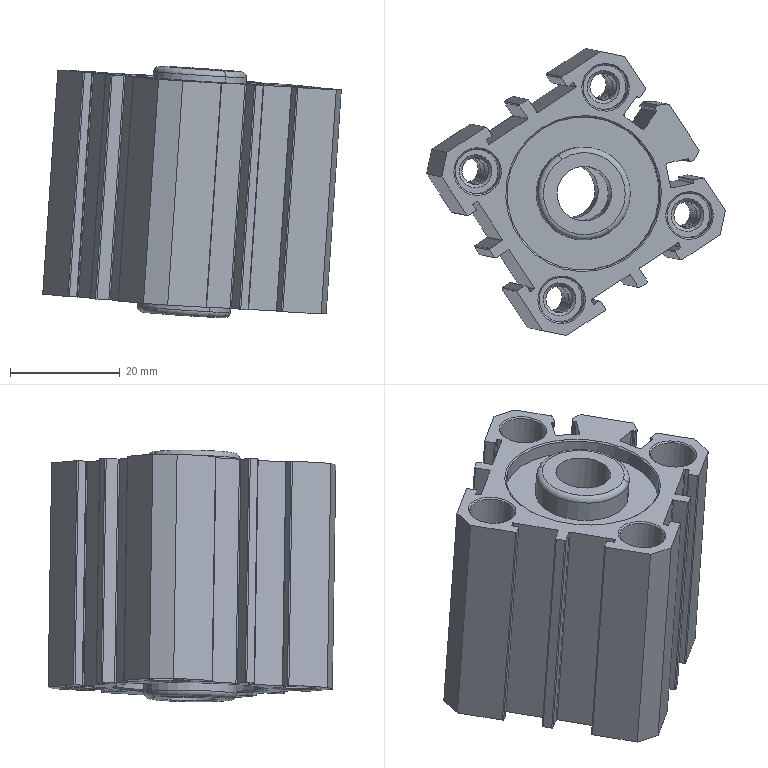Component | SolidWorks | SDAJ25x20-20B(00)+()-1_SDAJ-25x20_20b-1 | 1 solid | 245 faces | box 54.53 x 52.51 x 45.94 mm | volume 37343 mm3 | cylinder 111 | plane 86 | cone 44 | torus 4 | commonest cylinder face diameters 0.4 x46 8.2 x16 4.917 x16 4.6 x8 0.8 x7 17 x4 28 x4 4.134 x4
build123d program:
from build123d import *

# Parameters (mm, degrees)
BOSS_EXTRUDE1_DEPTH  = 41
LPATTERN1_COUNT      = 2
LPATTERN1_PITCH      = 28
LPATTERN1_COUNT_DIR2 = 2
LPATTERN1_PITCH_DIR2 = 28
LPATTERN2_COUNT      = 2
LPATTERN2_PITCH      = 28
LPATTERN2_COUNT_DIR2 = 2
LPATTERN2_PITCH_DIR2 = 28
HOLE1_D              = 4.134
HOLE1_DEPTH          = 6
HOLE1_CSINK_D        = 5
HOLE1_CSINK_ANGLE    = 90
HOLE1_TIP            = 1.193
HOLE2_D              = 4.134
HOLE2_DEPTH          = 6
HOLE2_CSINK_D        = 5
HOLE2_CSINK_ANGLE    = 90
HOLE2_TIP            = 1.193


with BuildPart() as part:
    # Sketch1 → Boss-Extrude1 (new body)
    with BuildSketch(Plane(origin=(0, 0, 0), x_dir=(0, 0, -1), z_dir=(1, 0, 0))):
        with BuildLine():
            Line((-20, 16.8), (-20, 8.4))
            ThreePointArc((-20, 8.4), (-19.941, 8.259), (-19.8, 8.2))
            Line((-19.8, 8.2), (-18.2, 8.2))
            ThreePointArc((-18.2, 8.2), (-18.059, 8.259), (-18, 8.4))
            Line((-18, 8.4), (-18, 9.4))
            ThreePointArc((-18, 9.4), (-17.941, 9.541), (-17.8, 9.6))
            Line((-17.8, 9.6), (-17.2, 9.6))
            ThreePointArc((-17.2, 9.6), (-17.059, 9.541), (-17, 9.4))
            Line((-17, 9.4), (-17, 1.2))
            ThreePointArc((-17, 1.2), (-17.059, 1.059), (-17.2, 1))
            Line((-17.2, 1), (-19.8, 1))
            ThreePointArc((-19.8, 1), (-19.941, 0.9414), (-20, 0.8))
            Line((-20, 0.8), (-20, -0.8))
            ThreePointArc((-20, -0.8), (-19.941, -0.9414), (-19.8, -1))
            Line((-19.8, -1), (-17.2, -1))
            ThreePointArc((-17.2, -1), (-17.059, -1.059), (-17, -1.2))
            Line((-17, -1.2), (-17, -9.4))
            ThreePointArc((-17, -9.4), (-17.059, -9.541), (-17.2, -9.6))
            Line((-17.2, -9.6), (-17.8, -9.6))
            ThreePointArc((-17.8, -9.6), (-17.941, -9.541), (-18, -9.4))
            Line((-18, -9.4), (-18, -8.4))
            ThreePointArc((-18, -8.4), (-18.059, -8.259), (-18.2, -8.2))
            Line((-18.2, -8.2), (-19.8, -8.2))
            ThreePointArc((-19.8, -8.2), (-19.941, -8.259), (-20, -8.4))
            Line((-20, -8.4), (-20, -16.8))
            Line((-20, -16.8), (-16.8, -20))
            Line((-16.8, -20), (-8.4, -20))
            ThreePointArc((-8.4, -20), (-8.259, -19.941), (-8.2, -19.8))
            Line((-8.2, -19.8), (-8.2, -18.2))
            ThreePointArc((-8.2, -18.2), (-8.259, -18.059), (-8.4, -18))
            Line((-8.4, -18), (-9.4, -18))
            ThreePointArc((-9.4, -18), (-9.541, -17.941), (-9.6, -17.8))
            Line((-9.6, -17.8), (-9.6, -17.2))
            ThreePointArc((-9.6, -17.2), (-9.541, -17.059), (-9.4, -17))
            Line((-9.4, -17), (-1.2, -17))
            ThreePointArc((-1.2, -17), (-1.059, -17.059), (-1, -17.2))
            Line((-1, -17.2), (-1, -19.8))
            ThreePointArc((-1, -19.8), (-0.9414, -19.941), (-0.8, -20))
            Line((-0.8, -20), (0.8, -20))
            ThreePointArc((0.8, -20), (0.9414, -19.941), (1, -19.8))
            Line((1, -19.8), (1, -17.2))
            ThreePointArc((1, -17.2), (1.059, -17.059), (1.2, -17))
            Line((1.2, -17), (9.4, -17))
            ThreePointArc((9.4, -17), (9.541, -17.059), (9.6, -17.2))
            Line((9.6, -17.2), (9.6, -17.8))
            ThreePointArc((9.6, -17.8), (9.541, -17.941), (9.4, -18))
            Line((9.4, -18), (8.4, -18))
            ThreePointArc((8.4, -18), (8.259, -18.059), (8.2, -18.2))
            Line((8.2, -18.2), (8.2, -19.8))
            ThreePointArc((8.2, -19.8), (8.259, -19.941), (8.4, -20))
            Line((8.4, -20), (16.8, -20))
            Line((16.8, -20), (20, -16.8))
            Line((20, -16.8), (20, -8.4))
            ThreePointArc((20, -8.4), (19.941, -8.259), (19.8, -8.2))
            Line((19.8, -8.2), (18.2, -8.2))
            ThreePointArc((18.2, -8.2), (18.059, -8.259), (18, -8.4))
            Line((18, -8.4), (18, -9.4))
            ThreePointArc((18, -9.4), (17.941, -9.541), (17.8, -9.6))
            Line((17.8, -9.6), (17.2, -9.6))
            ThreePointArc((17.2, -9.6), (17.059, -9.541), (17, -9.4))
            Line((17, -9.4), (17, -1.2))
            ThreePointArc((17, -1.2), (17.059, -1.059), (17.2, -1))
            Line((17.2, -1), (19.8, -1))
            ThreePointArc((19.8, -1), (19.941, -0.9414), (20, -0.8))
            Line((20, -0.8), (20, 0.8))
            ThreePointArc((20, 0.8), (19.941, 0.9414), (19.8, 1))
            Line((19.8, 1), (17.2, 1))
            ThreePointArc((17.2, 1), (17.059, 1.059), (17, 1.2))
            Line((17, 1.2), (17, 9.4))
            ThreePointArc((17, 9.4), (17.059, 9.541), (17.2, 9.6))
            Line((17.2, 9.6), (17.8, 9.6))
            ThreePointArc((17.8, 9.6), (17.941, 9.541), (18, 9.4))
            Line((18, 9.4), (18, 8.4))
            ThreePointArc((18, 8.4), (18.059, 8.259), (18.2, 8.2))
            Line((18.2, 8.2), (19.8, 8.2))
            ThreePointArc((19.8, 8.2), (19.941, 8.259), (20, 8.4))
            Line((20, 8.4), (20, 16.8))
            Line((20, 16.8), (16.8, 20))
            Line((16.8, 20), (9.978, 20))
            ThreePointArc((9.978, 20), (9.753, 19.931), (9.606, 19.747))
            Line((9.606, 19.747), (9.022, 18.264))
            ThreePointArc((9.022, 18.264), (9.024, 18.111), (9.134, 18.005))
            Line((9.134, 18.005), (9.321, 17.932))
            ThreePointArc((9.321, 17.932), (9.431, 17.825), (9.433, 17.672))
            Line((9.433, 17.672), (8.077, 14.23))
            ThreePointArc((8.077, 14.23), (7.865, 14.01), (7.559, 14.004))
            Line((7.559, 14.004), (4.023, 15.397))
            ThreePointArc((4.023, 15.397), (3.803, 15.61), (3.797, 15.916))
            Line((3.797, 15.916), (5.153, 19.358))
            ThreePointArc((5.153, 19.358), (5.26, 19.468), (5.413, 19.471))
            Line((5.413, 19.471), (5.581, 19.405))
            ThreePointArc((5.581, 19.405), (5.742, 19.411), (5.846, 19.535))
            Line((5.846, 19.535), (6.039, 20.2))
            Line((6.039, 20.2), (5, 22))
            Line((5, 22), (-5, 22))
            Line((-5, 22), (-6.039, 20.2))
            Line((-6.039, 20.2), (-5.846, 19.535))
            ThreePointArc((-5.846, 19.535), (-5.742, 19.411), (-5.581, 19.405))
            Line((-5.581, 19.405), (-5.413, 19.471))
            ThreePointArc((-5.413, 19.471), (-5.26, 19.468), (-5.153, 19.358))
            Line((-5.153, 19.358), (-3.797, 15.916))
            ThreePointArc((-3.797, 15.916), (-3.803, 15.61), (-4.023, 15.397))
            Line((-4.023, 15.397), (-7.559, 14.004))
            ThreePointArc((-7.559, 14.004), (-7.865, 14.01), (-8.077, 14.23))
            Line((-8.077, 14.23), (-9.433, 17.672))
            ThreePointArc((-9.433, 17.672), (-9.431, 17.825), (-9.321, 17.932))
            Line((-9.321, 17.932), (-9.134, 18.005))
            ThreePointArc((-9.134, 18.005), (-9.024, 18.111), (-9.022, 18.264))
            Line((-9.022, 18.264), (-9.606, 19.747))
            ThreePointArc((-9.606, 19.747), (-9.753, 19.931), (-9.978, 20))
            Line((-9.978, 20), (-16.8, 20))
            Line((-16.8, 20), (-20, 16.8))
        make_face()
    extrude(amount=BOSS_EXTRUDE1_DEPTH)

    # Sketch2 → Cut-Revolve1 (revolve, cut)
    with BuildSketch(Plane.XY.offset(14), mode=Mode.PRIVATE) as cut_revolve1_sk:
        Polygon((0, -14), (0, -9.65), (0.25, -9.9), (5.5, -9.9), (5.5, -11), (6.042, -11.541), (15, -11.541), (15, -11.7), (20.5, -11.7), (20.5, -14), align=None)
    cut_revolve1 = revolve(cut_revolve1_sk.sketch.rotate(Axis((20.5, -14, 14), (-1, 0, 0)), 270), axis=Axis((20.5, -14, 14), (-1, 0, 0)), mode=Mode.SUBTRACT)

    # LPattern1: Cut-Revolve1 2 × 2
    with Locations(*[(0, j * LPATTERN1_PITCH_DIR2, -i * LPATTERN1_PITCH) for i in range(LPATTERN1_COUNT) for j in range(LPATTERN1_COUNT_DIR2) if (i, j) != (0, 0)]):
        add(cut_revolve1, mode=Mode.SUBTRACT)

    # Sketch4 → Cut-Revolve2 (revolve, cut)
    with BuildSketch(Plane.XY.offset(14), mode=Mode.PRIVATE) as cut_revolve2_sk:
        Polygon((20.5, -14), (20.5, -11.7), (26, -11.7), (26, -11.541), (34.959, -11.541), (35.5, -11), (35.5, -9.9), (40.75, -9.9), (41, -9.65), (41, -14), align=None)
    cut_revolve2 = revolve(cut_revolve2_sk.sketch.rotate(Axis((41, -14, 14), (-1, 0, 0)), 270), axis=Axis((41, -14, 14), (-1, 0, 0)), mode=Mode.SUBTRACT)

    # LPattern2: Cut-Revolve2 2 × 2
    with Locations(*[(0, j * LPATTERN2_PITCH_DIR2, -i * LPATTERN2_PITCH) for i in range(LPATTERN2_COUNT) for j in range(LPATTERN2_COUNT_DIR2) if (i, j) != (0, 0)]):
        add(cut_revolve2, mode=Mode.SUBTRACT)

    # Hole1
    with Locations(Plane(origin=(0, 22, 0), x_dir=(1, 0, 0), z_dir=(0, 1, 0))):
        with Locations((8, 0)):
            CounterSinkHole(HOLE1_D / 2, HOLE1_CSINK_D / 2, depth=HOLE1_DEPTH, counter_sink_angle=HOLE1_CSINK_ANGLE)
            with Locations((0, 0, -(HOLE1_DEPTH + HOLE1_TIP / 2))):  # 120° drill point
                Cone(0, HOLE1_D / 2, HOLE1_TIP, mode=Mode.SUBTRACT)

    # Hole2
    with Locations(Plane(origin=(0, 22, 0), x_dir=(1, 0, 0), z_dir=(0, 1, 0))):
        with Locations((33, 0)):
            CounterSinkHole(HOLE2_D / 2, HOLE2_CSINK_D / 2, depth=HOLE2_DEPTH, counter_sink_angle=HOLE2_CSINK_ANGLE)
            with Locations((0, 0, -(HOLE2_DEPTH + HOLE2_TIP / 2))):  # 120° drill point
                Cone(0, HOLE2_D / 2, HOLE2_TIP, mode=Mode.SUBTRACT)

    # Sketch10 → Cut-Revolve3 (revolve, cut)
    with BuildSketch(Plane.XY, mode=Mode.PRIVATE) as cut_revolve3_sk:
        Polygon((0, 0), (0, 5), (7, 5), (7, 12.5), (34, 12.5), (34, 5), (41, 5), (41, 0), align=None)
    revolve(cut_revolve3_sk.sketch.rotate(Axis((41, 0, 0), (-1, 0, 0)), 270), axis=Axis((41, 0, 0), (-1, 0, 0)), mode=Mode.SUBTRACT)

    # Sketch11 → Cut-Revolve4 (revolve, cut)
    with BuildSketch(Plane.XY, mode=Mode.PRIVATE) as cut_revolve4_sk:
        Polygon((0, 0), (0, 14.3), (0.3, 14), (2.8, 14), (2.8, 0), align=None)
    revolve(cut_revolve4_sk.sketch.rotate(Axis((2.8, 0, 0), (-1, 0, 0)), 270), axis=Axis((2.8, 0, 0), (-1, 0, 0)), mode=Mode.SUBTRACT)

    # Sketch12 → Revolve1 (revolve)
    with BuildSketch(Plane.XY, mode=Mode.PRIVATE) as revolve1_sk:
        with BuildLine():
            Line((-2, 7.5), (-2, 5))
            Line((-2, 5), (2.8, 5))
            Line((2.8, 5), (2.8, 8.5))
            Line((2.8, 8.5), (-1, 8.5))
            ThreePointArc((-1, 8.5), (-1.707, 8.207), (-2, 7.5))
        make_face()
    revolve(revolve1_sk.sketch.rotate(Axis((2.8, 0, 0), (-1, 0, 0)), 270), axis=Axis((2.8, 0, 0), (-1, 0, 0)))

    # Sketch13 → Cut-Revolve5 (revolve, cut)
    with BuildSketch(Plane.XY, mode=Mode.PRIVATE) as cut_revolve5_sk:
        Polygon((38.2, 0), (38.2, 14), (40.75, 14), (41, 14.25), (41, 0), align=None)
    revolve(cut_revolve5_sk.sketch.rotate(Axis((41, 0, 0), (-1, 0, 0)), 270), axis=Axis((41, 0, 0), (-1, 0, 0)), mode=Mode.SUBTRACT)

    # Sketch14 → Revolve2 (revolve)
    with BuildSketch(Plane.XY, mode=Mode.PRIVATE) as revolve2_sk:
        with BuildLine():
            Line((38.2, 5), (43, 5))
            Line((43, 5), (43, 7.5))
            ThreePointArc((43, 7.5), (42.707, 8.207), (42, 8.5))
            Line((42, 8.5), (38.2, 8.5))
            Line((38.2, 8.5), (38.2, 5))
        make_face()
    revolve(revolve2_sk.sketch.rotate(Axis((43, 0, 0), (-1, 0, 0)), 270), axis=Axis((43, 0, 0), (-1, 0, 0)))


solid = part.part

# Placed as in the assembly
solid = solid.moved(Location((-91.288, 142.459, 793.096), (-86.571, -33.197, -85.373)))